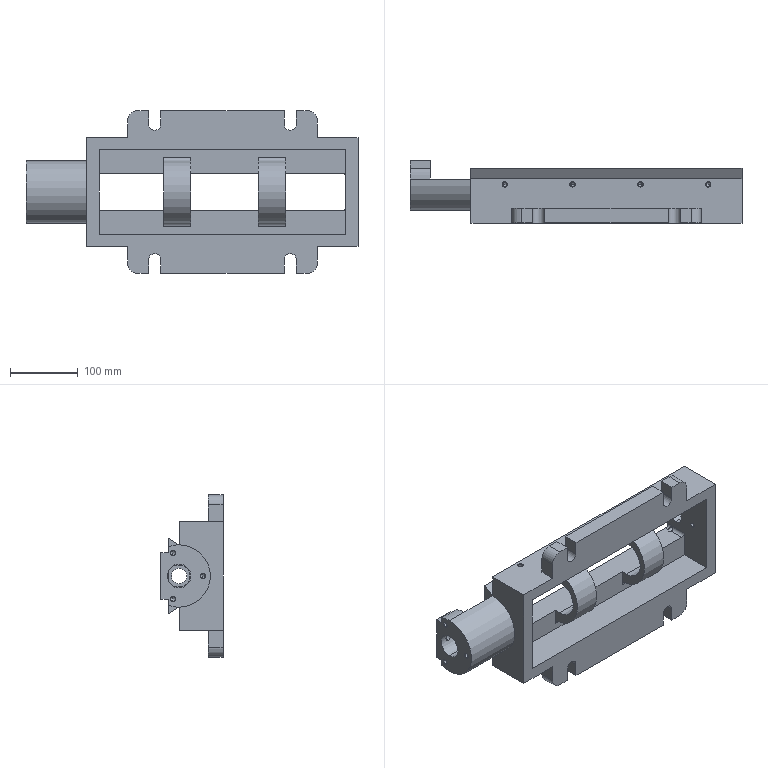Component | SolidWorks | 4Base-1 | 1 solid | 168 faces | volume 2787112 mm3 | cylinder 61 | plane 54 | cone 53 | commonest cylinder face diameters 6.8 x28 10 x6 18 x6 92 x5 30 x4 12 x4 23 x2 35 x2